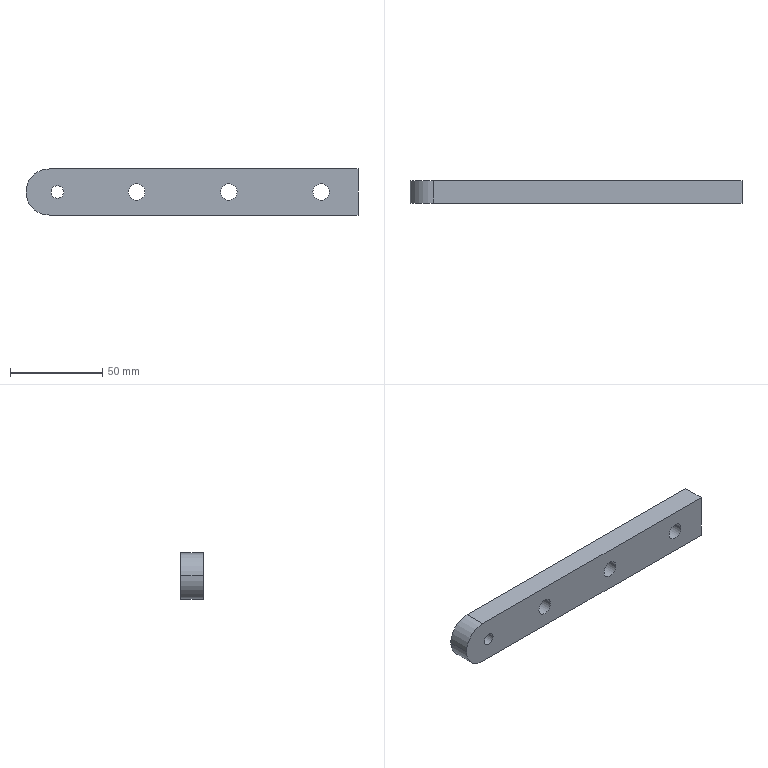Component | SolidWorks | CuttingDie-1_LocatingStrip-1 | 1 solid | 21 faces | box 180 x 12 x 25 mm | volume 49435 mm3 | cylinder 10 | cone 6 | plane 5 | commonest cylinder face diameters 9 x6 6.8 x2 25 x2
build123d program:
from build123d import *

# Parameters (mm, degrees)
SKETCH1_W                                         = 25
SKETCH1_H                                         = 12
BOSS_EXTRUDE1_DEPTH                               = 90
FILLET1_RADIUS                                    = 12.5
FILLET1_LENGTH                                    = 12
HOLE_SIZE_ACCORDING_TO_TYPE_1_OF_HEXA_D           = 9
HOLE_SIZE_ACCORDING_TO_TYPE_1_OF_HEXA_CSINK_D     = 17.6
HOLE_SIZE_ACCORDING_TO_TYPE_1_OF_HEXA_CSINK_ANGLE = 90
M8_TAPPED_HOLE1_D                                 = 6.8


with BuildPart() as part:
    # Sketch1 → Boss-Extrude1 (new, symmetric)
    with BuildSketch(Plane.XY):
        Rectangle(SKETCH1_W, SKETCH1_H)
    extrude(amount=BOSS_EXTRUDE1_DEPTH, both=True)

    # Fillet1: full round fillet: the end face becomes a half cylinder, R = half its width
    fillet1_face = Plane((0, 0, 90), x_dir=(0, 1, 0), z_dir=(0, 0, 1))  # on the end face: x along it, z out of the body
    fillet1_slab = fillet1_face.offset(-FILLET1_RADIUS / 2) * Box(FILLET1_LENGTH, 2 * FILLET1_RADIUS, FILLET1_RADIUS, mode=Mode.PRIVATE)  # the body's end, R deep
    fillet1_round = Plane((0, 0, 77.5), x_dir=(0, 0, 1), z_dir=(0, 1, 0)) * Cylinder(FILLET1_RADIUS, FILLET1_LENGTH, mode=Mode.PRIVATE)  # its axis R under the face
    add(fillet1_slab - fillet1_round, mode=Mode.SUBTRACT)

    # Hole Size _ according to_ Type 1 of Hexa (through all)
    with Locations(Plane(origin=(0, 6, 0), x_dir=(1, 0, 0), z_dir=(0, 1, 0))):
        with Locations((0, 70), (0, 20), (0, -30)):
            CounterSinkHole(HOLE_SIZE_ACCORDING_TO_TYPE_1_OF_HEXA_D / 2, HOLE_SIZE_ACCORDING_TO_TYPE_1_OF_HEXA_CSINK_D / 2, counter_sink_angle=HOLE_SIZE_ACCORDING_TO_TYPE_1_OF_HEXA_CSINK_ANGLE)

    # M8 Tapped Hole1 (through all)
    with Locations(Plane(origin=(0, 6, 0), x_dir=(1, 0, 0), z_dir=(0, 1, 0))):
        with Locations((0, -73)):
            Hole(M8_TAPPED_HOLE1_D / 2)


solid = part.part

# Placed as in the assembly
solid = solid.moved(Location((-441.772, -450.766, 1107), (0, -90, 0)))
STEP:
#1=COLOUR_RGB('',0.7922,0.8196,0.9333);
#2=FILL_AREA_STYLE_COLOUR('',#1);
#3=FILL_AREA_STYLE('',(#2));
#4=SURFACE_STYLE_FILL_AREA(#3);
#5=SURFACE_SIDE_STYLE('',(#4));
#6=SURFACE_STYLE_USAGE(.BOTH.,#5);
#7=PRESENTATION_STYLE_ASSIGNMENT((#6));
#8=CARTESIAN_POINT('',(-20.133,-17.983,43.583));
#9=VERTEX_POINT('',#8);
#10=CARTESIAN_POINT('',(-20.4,-17.983,43.583));
#11=VERTEX_POINT('',#10);
#12=CARTESIAN_POINT('',(-20.267,-17.983,43.583));
#13=DIRECTION('',(-0.,1.,0.));
#14=DIRECTION('',(-1.,0.,0.));
#15=AXIS2_PLACEMENT_3D('',#12,#13,#14);
#16=CIRCLE('',#15,0.1339);
#17=EDGE_CURVE('',#9,#11,#16,.T.);
#18=ORIENTED_EDGE('',*,*,#17,.F.);
#19=CARTESIAN_POINT('',(-20.133,-17.51,43.583));
#20=VERTEX_POINT('',#19);
#21=CARTESIAN_POINT('',(-20.133,-17.51,43.583));
#22=DIRECTION('',(-0.,1.,0.));
#23=VECTOR('',#22,39.37);
#24=LINE('',#21,#23);
#25=EDGE_CURVE('',#9,#20,#24,.T.);
#26=ORIENTED_EDGE('',*,*,#25,.T.);
#27=CARTESIAN_POINT('',(-20.4,-17.51,43.583));
#28=VERTEX_POINT('',#27);
#29=CARTESIAN_POINT('',(-20.267,-17.51,43.583));
#30=DIRECTION('',(-0.,1.,0.));
#31=DIRECTION('',(-1.,0.,0.));
#32=AXIS2_PLACEMENT_3D('',#29,#30,#31);
#33=CIRCLE('',#32,0.1339);
#34=EDGE_CURVE('',#20,#28,#33,.T.);
#35=ORIENTED_EDGE('',*,*,#34,.T.);
#36=CARTESIAN_POINT('',(-20.4,-17.51,43.583));
#37=DIRECTION('',(-0.,1.,0.));
#38=VECTOR('',#37,39.37);
#39=LINE('',#36,#38);
#40=EDGE_CURVE('',#11,#28,#39,.T.);
#41=ORIENTED_EDGE('',*,*,#40,.F.);
#42=EDGE_LOOP('',(#18,#26,#35,#41));
#43=FACE_OUTER_BOUND('',#42,.T.);
#44=CARTESIAN_POINT('',(-20.267,-17.51,43.583));
#45=DIRECTION('',(-0.,1.,0.));
#46=DIRECTION('',(-1.,0.,0.));
#47=AXIS2_PLACEMENT_3D('',#44,#45,#46);
#48=CYLINDRICAL_SURFACE('',#47,0.1339);
#49=ADVANCED_FACE('',(#43),#48,.F.);
#50=CARTESIAN_POINT('',(-14.46,-17.68,43.583));
#51=VERTEX_POINT('',#50);
#52=CARTESIAN_POINT('',(-14.814,-17.68,43.583));
#53=VERTEX_POINT('',#52);
#54=CARTESIAN_POINT('',(-14.637,-17.68,43.583));
#55=DIRECTION('',(-0.,1.,0.));
#56=DIRECTION('',(-1.,0.,0.));
#57=AXIS2_PLACEMENT_3D('',#54,#55,#56);
#58=CIRCLE('',#57,0.1772);
#59=EDGE_CURVE('',#51,#53,#58,.T.);
#60=ORIENTED_EDGE('',*,*,#59,.F.);
#61=CARTESIAN_POINT('',(-14.29,-17.51,43.583));
#62=VERTEX_POINT('',#61);
#63=CARTESIAN_POINT('',(-14.29,-17.51,43.583));
#64=DIRECTION('',(0.7071,0.7071,0.));
#65=VECTOR('',#64,39.37);
#66=LINE('',#63,#65);
#67=EDGE_CURVE('',#51,#62,#66,.T.);
#68=ORIENTED_EDGE('',*,*,#67,.T.);
#69=CARTESIAN_POINT('',(-14.983,-17.51,43.583));
#70=VERTEX_POINT('',#69);
#71=CARTESIAN_POINT('',(-14.637,-17.51,43.583));
#72=DIRECTION('',(-0.,1.,0.));
#73=DIRECTION('',(-1.,0.,0.));
#74=AXIS2_PLACEMENT_3D('',#71,#72,#73);
#75=CIRCLE('',#74,0.3465);
#76=EDGE_CURVE('',#62,#70,#75,.T.);
#77=ORIENTED_EDGE('',*,*,#76,.T.);
#78=CARTESIAN_POINT('',(-14.983,-17.51,43.583));
#79=DIRECTION('',(-0.7071,0.7071,-0.));
#80=VECTOR('',#79,39.37);
#81=LINE('',#78,#80);
#82=EDGE_CURVE('',#53,#70,#81,.T.);
#83=ORIENTED_EDGE('',*,*,#82,.F.);
#84=EDGE_LOOP('',(#60,#68,#77,#83));
#85=FACE_OUTER_BOUND('',#84,.T.);
#86=CARTESIAN_POINT('',(-14.637,-17.51,43.583));
#87=DIRECTION('',(-0.,1.,0.));
#88=DIRECTION('',(-1.,0.,0.));
#89=AXIS2_PLACEMENT_3D('',#86,#87,#88);
#90=CONICAL_SURFACE('',#89,0.3465,0.7854);
#91=ADVANCED_FACE('',(#85),#90,.F.);
#92=CARTESIAN_POINT('',(-14.46,-17.983,43.583));
#93=VERTEX_POINT('',#92);
#94=CARTESIAN_POINT('',(-14.814,-17.983,43.583));
#95=VERTEX_POINT('',#94);
#96=CARTESIAN_POINT('',(-14.637,-17.983,43.583));
#97=DIRECTION('',(-0.,1.,0.));
#98=DIRECTION('',(-1.,0.,0.));
#99=AXIS2_PLACEMENT_3D('',#96,#97,#98);
#100=CIRCLE('',#99,0.1772);
#101=EDGE_CURVE('',#93,#95,#100,.T.);
#102=ORIENTED_EDGE('',*,*,#101,.F.);
#103=CARTESIAN_POINT('',(-14.46,-17.51,43.583));
#104=DIRECTION('',(-0.,1.,0.));
#105=VECTOR('',#104,39.37);
#106=LINE('',#103,#105);
#107=EDGE_CURVE('',#93,#51,#106,.T.);
#108=ORIENTED_EDGE('',*,*,#107,.T.);
#109=ORIENTED_EDGE('',*,*,#59,.T.);
#110=CARTESIAN_POINT('',(-14.814,-17.51,43.583));
#111=DIRECTION('',(-0.,1.,0.));
#112=VECTOR('',#111,39.37);
#113=LINE('',#110,#112);
#114=EDGE_CURVE('',#95,#53,#113,.T.);
#115=ORIENTED_EDGE('',*,*,#114,.F.);
#116=EDGE_LOOP('',(#102,#108,#109,#115));
#117=FACE_OUTER_BOUND('',#116,.T.);
#118=CARTESIAN_POINT('',(-14.637,-17.51,43.583));
#119=DIRECTION('',(-0.,1.,0.));
#120=DIRECTION('',(-1.,0.,0.));
#121=AXIS2_PLACEMENT_3D('',#118,#119,#120);
#122=CYLINDRICAL_SURFACE('',#121,0.1772);
#123=ADVANCED_FACE('',(#117),#122,.F.);
#124=CARTESIAN_POINT('',(-16.428,-17.68,43.583));
#125=VERTEX_POINT('',#124);
#126=CARTESIAN_POINT('',(-16.782,-17.68,43.583));
#127=VERTEX_POINT('',#126);
#128=CARTESIAN_POINT('',(-16.605,-17.68,43.583));
#129=DIRECTION('',(-0.,1.,0.));
#130=DIRECTION('',(-1.,0.,0.));
#131=AXIS2_PLACEMENT_3D('',#128,#129,#130);
#132=CIRCLE('',#131,0.1772);
#133=EDGE_CURVE('',#125,#127,#132,.T.);
#134=ORIENTED_EDGE('',*,*,#133,.F.);
#135=CARTESIAN_POINT('',(-16.259,-17.51,43.583));
#136=VERTEX_POINT('',#135);
#137=CARTESIAN_POINT('',(-16.259,-17.51,43.583));
#138=DIRECTION('',(0.7071,0.7071,0.));
#139=VECTOR('',#138,39.37);
#140=LINE('',#137,#139);
#141=EDGE_CURVE('',#125,#136,#140,.T.);
#142=ORIENTED_EDGE('',*,*,#141,.T.);
#143=CARTESIAN_POINT('',(-16.952,-17.51,43.583));
#144=VERTEX_POINT('',#143);
#145=CARTESIAN_POINT('',(-16.605,-17.51,43.583));
#146=DIRECTION('',(-0.,1.,0.));
#147=DIRECTION('',(-1.,0.,0.));
#148=AXIS2_PLACEMENT_3D('',#145,#146,#147);
#149=CIRCLE('',#148,0.3465);
#150=EDGE_CURVE('',#136,#144,#149,.T.);
#151=ORIENTED_EDGE('',*,*,#150,.T.);
#152=CARTESIAN_POINT('',(-16.952,-17.51,43.583));
#153=DIRECTION('',(-0.7071,0.7071,-0.));
#154=VECTOR('',#153,39.37);
#155=LINE('',#152,#154);
#156=EDGE_CURVE('',#127,#144,#155,.T.);
#157=ORIENTED_EDGE('',*,*,#156,.F.);
#158=EDGE_LOOP('',(#134,#142,#151,#157));
#159=FACE_OUTER_BOUND('',#158,.T.);
#160=CARTESIAN_POINT('',(-16.605,-17.51,43.583));
#161=DIRECTION('',(-0.,1.,0.));
#162=DIRECTION('',(-1.,0.,0.));
#163=AXIS2_PLACEMENT_3D('',#160,#161,#162);
#164=CONICAL_SURFACE('',#163,0.3465,0.7854);
#165=ADVANCED_FACE('',(#159),#164,.F.);
#166=CARTESIAN_POINT('',(-16.428,-17.983,43.583));
#167=VERTEX_POINT('',#166);
#168=CARTESIAN_POINT('',(-16.782,-17.983,43.583));
#169=VERTEX_POINT('',#168);
#170=CARTESIAN_POINT('',(-16.605,-17.983,43.583));
#171=DIRECTION('',(-0.,1.,0.));
#172=DIRECTION('',(-1.,0.,0.));
#173=AXIS2_PLACEMENT_3D('',#170,#171,#172);
#174=CIRCLE('',#173,0.1772);
#175=EDGE_CURVE('',#167,#169,#174,.T.);
#176=ORIENTED_EDGE('',*,*,#175,.F.);
#177=CARTESIAN_POINT('',(-16.428,-17.51,43.583));
#178=DIRECTION('',(-0.,1.,0.));
#179=VECTOR('',#178,39.37);
#180=LINE('',#177,#179);
#181=EDGE_CURVE('',#167,#125,#180,.T.);
#182=ORIENTED_EDGE('',*,*,#181,.T.);
#183=ORIENTED_EDGE('',*,*,#133,.T.);
#184=CARTESIAN_POINT('',(-16.782,-17.51,43.583));
#185=DIRECTION('',(-0.,1.,0.));
#186=VECTOR('',#185,39.37);
#187=LINE('',#184,#186);
#188=EDGE_CURVE('',#169,#127,#187,.T.);
#189=ORIENTED_EDGE('',*,*,#188,.F.);
#190=EDGE_LOOP('',(#176,#182,#183,#189));
#191=FACE_OUTER_BOUND('',#190,.T.);
#192=CARTESIAN_POINT('',(-16.605,-17.51,43.583));
#193=DIRECTION('',(-0.,1.,0.));
#194=DIRECTION('',(-1.,0.,0.));
#195=AXIS2_PLACEMENT_3D('',#192,#193,#194);
#196=CYLINDRICAL_SURFACE('',#195,0.1772);
#197=ADVANCED_FACE('',(#191),#196,.F.);
#198=CARTESIAN_POINT('',(-18.397,-17.68,43.583));
#199=VERTEX_POINT('',#198);
#200=CARTESIAN_POINT('',(-18.751,-17.68,43.583));
#201=VERTEX_POINT('',#200);
#202=CARTESIAN_POINT('',(-18.574,-17.68,43.583));
#203=DIRECTION('',(-0.,1.,0.));
#204=DIRECTION('',(-1.,0.,0.));
#205=AXIS2_PLACEMENT_3D('',#202,#203,#204);
#206=CIRCLE('',#205,0.1772);
#207=EDGE_CURVE('',#199,#201,#206,.T.);
#208=ORIENTED_EDGE('',*,*,#207,.F.);
#209=CARTESIAN_POINT('',(-18.227,-17.51,43.583));
#210=VERTEX_POINT('',#209);
#211=CARTESIAN_POINT('',(-18.227,-17.51,43.583));
#212=DIRECTION('',(0.7071,0.7071,0.));
#213=VECTOR('',#212,39.37);
#214=LINE('',#211,#213);
#215=EDGE_CURVE('',#199,#210,#214,.T.);
#216=ORIENTED_EDGE('',*,*,#215,.T.);
#217=CARTESIAN_POINT('',(-18.92,-17.51,43.583));
#218=VERTEX_POINT('',#217);
#219=CARTESIAN_POINT('',(-18.574,-17.51,43.583));
#220=DIRECTION('',(-0.,1.,0.));
#221=DIRECTION('',(-1.,0.,0.));
#222=AXIS2_PLACEMENT_3D('',#219,#220,#221);
#223=CIRCLE('',#222,0.3465);
#224=EDGE_CURVE('',#210,#218,#223,.T.);
#225=ORIENTED_EDGE('',*,*,#224,.T.);
#226=CARTESIAN_POINT('',(-18.92,-17.51,43.583));
#227=DIRECTION('',(-0.7071,0.7071,-0.));
#228=VECTOR('',#227,39.37);
#229=LINE('',#226,#228);
#230=EDGE_CURVE('',#201,#218,#229,.T.);
#231=ORIENTED_EDGE('',*,*,#230,.F.);
#232=EDGE_LOOP('',(#208,#216,#225,#231));
#233=FACE_OUTER_BOUND('',#232,.T.);
#234=CARTESIAN_POINT('',(-18.574,-17.51,43.583));
#235=DIRECTION('',(-0.,1.,0.));
#236=DIRECTION('',(-1.,0.,0.));
#237=AXIS2_PLACEMENT_3D('',#234,#235,#236);
#238=CONICAL_SURFACE('',#237,0.3465,0.7854);
#239=ADVANCED_FACE('',(#233),#238,.F.);
#240=CARTESIAN_POINT('',(-18.397,-17.983,43.583));
#241=VERTEX_POINT('',#240);
#242=CARTESIAN_POINT('',(-18.751,-17.983,43.583));
#243=VERTEX_POINT('',#242);
#244=CARTESIAN_POINT('',(-18.574,-17.983,43.583));
#245=DIRECTION('',(-0.,1.,0.));
#246=DIRECTION('',(-1.,0.,0.));
#247=AXIS2_PLACEMENT_3D('',#244,#245,#246);
#248=CIRCLE('',#247,0.1772);
#249=EDGE_CURVE('',#241,#243,#248,.T.);
#250=ORIENTED_EDGE('',*,*,#249,.F.);
#251=CARTESIAN_POINT('',(-18.397,-17.51,43.583));
#252=DIRECTION('',(-0.,1.,0.));
#253=VECTOR('',#252,39.37);
#254=LINE('',#251,#253);
#255=EDGE_CURVE('',#241,#199,#254,.T.);
#256=ORIENTED_EDGE('',*,*,#255,.T.);
#257=ORIENTED_EDGE('',*,*,#207,.T.);
#258=CARTESIAN_POINT('',(-18.751,-17.51,43.583));
#259=DIRECTION('',(-0.,1.,0.));
#260=VECTOR('',#259,39.37);
#261=LINE('',#258,#260);
#262=EDGE_CURVE('',#243,#201,#261,.T.);
#263=ORIENTED_EDGE('',*,*,#262,.F.);
#264=EDGE_LOOP('',(#250,#256,#257,#263));
#265=FACE_OUTER_BOUND('',#264,.T.);
#266=CARTESIAN_POINT('',(-18.574,-17.51,43.583));
#267=DIRECTION('',(-0.,1.,0.));
#268=DIRECTION('',(-1.,0.,0.));
#269=AXIS2_PLACEMENT_3D('',#266,#267,#268);
#270=CYLINDRICAL_SURFACE('',#269,0.1772);
#271=ADVANCED_FACE('',(#265),#270,.F.);
#272=CARTESIAN_POINT('',(-20.936,-17.983,43.583));
#273=VERTEX_POINT('',#272);
#274=CARTESIAN_POINT('',(-20.444,-17.983,43.091));
#275=VERTEX_POINT('',#274);
#276=CARTESIAN_POINT('',(-20.444,-17.983,43.583));
#277=DIRECTION('',(0.,-1.,0.));
#278=DIRECTION('',(0.,0.,-1.));
#279=AXIS2_PLACEMENT_3D('',#276,#277,#278);
#280=CIRCLE('',#279,0.4921);
#281=EDGE_CURVE('',#273,#275,#280,.T.);
#282=ORIENTED_EDGE('',*,*,#281,.F.);
#283=CARTESIAN_POINT('',(-20.936,-17.51,43.583));
#284=VERTEX_POINT('',#283);
#285=CARTESIAN_POINT('',(-20.936,-17.51,43.583));
#286=DIRECTION('',(-0.,1.,0.));
#287=VECTOR('',#286,39.37);
#288=LINE('',#285,#287);
#289=EDGE_CURVE('',#273,#284,#288,.T.);
#290=ORIENTED_EDGE('',*,*,#289,.T.);
#291=CARTESIAN_POINT('',(-20.444,-17.51,43.091));
#292=VERTEX_POINT('',#291);
#293=CARTESIAN_POINT('',(-20.444,-17.51,43.583));
#294=DIRECTION('',(-0.,1.,0.));
#295=DIRECTION('',(1.,0.,0.));
#296=AXIS2_PLACEMENT_3D('',#293,#294,#295);
#297=CIRCLE('',#296,0.4921);
#298=EDGE_CURVE('',#292,#284,#297,.T.);
#299=ORIENTED_EDGE('',*,*,#298,.F.);
#300=CARTESIAN_POINT('',(-20.444,-17.51,43.091));
#301=DIRECTION('',(-0.,1.,0.));
#302=VECTOR('',#301,39.37);
#303=LINE('',#300,#302);
#304=EDGE_CURVE('',#275,#292,#303,.T.);
#305=ORIENTED_EDGE('',*,*,#304,.F.);
#306=EDGE_LOOP('',(#282,#290,#299,#305));
#307=FACE_OUTER_BOUND('',#306,.T.);
#308=CARTESIAN_POINT('',(-20.444,-17.51,43.583));
#309=DIRECTION('',(-0.,1.,0.));
#310=DIRECTION('',(-1.,0.,0.));
#311=AXIS2_PLACEMENT_3D('',#308,#309,#310);
#312=CYLINDRICAL_SURFACE('',#311,0.4921);
#313=ADVANCED_FACE('',(#307),#312,.T.);
#314=ORIENTED_EDGE('',*,*,#289,.F.);
#315=CARTESIAN_POINT('',(-20.444,-17.983,44.075));
#316=VERTEX_POINT('',#315);
#317=CARTESIAN_POINT('',(-20.444,-17.983,43.583));
#318=DIRECTION('',(0.,-1.,0.));
#319=DIRECTION('',(0.,0.,-1.));
#320=AXIS2_PLACEMENT_3D('',#317,#318,#319);
#321=CIRCLE('',#320,0.4921);
#322=EDGE_CURVE('',#316,#273,#321,.T.);
#323=ORIENTED_EDGE('',*,*,#322,.F.);
#324=CARTESIAN_POINT('',(-20.444,-17.51,44.075));
#325=VERTEX_POINT('',#324);
#326=CARTESIAN_POINT('',(-20.444,-17.51,44.075));
#327=DIRECTION('',(0.,-1.,-0.));
#328=VECTOR('',#327,39.37);
#329=LINE('',#326,#328);
#330=EDGE_CURVE('',#325,#316,#329,.T.);
#331=ORIENTED_EDGE('',*,*,#330,.F.);
#332=CARTESIAN_POINT('',(-20.444,-17.51,43.583));
#333=DIRECTION('',(-0.,1.,0.));
#334=DIRECTION('',(1.,0.,0.));
#335=AXIS2_PLACEMENT_3D('',#332,#333,#334);
#336=CIRCLE('',#335,0.4921);
#337=EDGE_CURVE('',#284,#325,#336,.T.);
#338=ORIENTED_EDGE('',*,*,#337,.F.);
#339=EDGE_LOOP('',(#314,#323,#331,#338));
#340=FACE_OUTER_BOUND('',#339,.T.);
#341=CARTESIAN_POINT('',(-20.444,-17.51,43.583));
#342=DIRECTION('',(-0.,1.,0.));
#343=DIRECTION('',(-1.,0.,0.));
#344=AXIS2_PLACEMENT_3D('',#341,#342,#343);
#345=CYLINDRICAL_SURFACE('',#344,0.4921);
#346=ADVANCED_FACE('',(#340),#345,.T.);
#347=CARTESIAN_POINT('',(-13.849,-17.983,43.091));
#348=VERTEX_POINT('',#347);
#349=CARTESIAN_POINT('',(-20.936,-17.983,43.091));
#350=DIRECTION('',(1.,0.,0.));
#351=VECTOR('',#350,39.37);
#352=LINE('',#349,#351);
#353=EDGE_CURVE('',#275,#348,#352,.T.);
#354=ORIENTED_EDGE('',*,*,#353,.F.);
#355=ORIENTED_EDGE('',*,*,#304,.T.);
#356=CARTESIAN_POINT('',(-13.849,-17.51,43.091));
#357=VERTEX_POINT('',#356);
#358=CARTESIAN_POINT('',(-20.936,-17.51,43.091));
#359=DIRECTION('',(1.,0.,0.));
#360=VECTOR('',#359,39.37);
#361=LINE('',#358,#360);
#362=EDGE_CURVE('',#292,#357,#361,.T.);
#363=ORIENTED_EDGE('',*,*,#362,.T.);
#364=CARTESIAN_POINT('',(-13.849,-17.983,43.091));
#365=DIRECTION('',(0.,-1.,-0.));
#366=VECTOR('',#365,39.37);
#367=LINE('',#364,#366);
#368=EDGE_CURVE('',#357,#348,#367,.T.);
#369=ORIENTED_EDGE('',*,*,#368,.T.);
#370=EDGE_LOOP('',(#354,#355,#363,#369));
#371=FACE_OUTER_BOUND('',#370,.T.);
#372=CARTESIAN_POINT('',(-20.936,-17.983,43.091));
#373=DIRECTION('',(-0.,-0.,1.));
#374=DIRECTION('',(1.,0.,0.));
#375=AXIS2_PLACEMENT_3D('',#372,#373,#374);
#376=PLANE('',#375);
#377=ADVANCED_FACE('',(#371),#376,.F.);
#378=CARTESIAN_POINT('',(-20.267,-17.983,43.583));
#379=DIRECTION('',(-0.,1.,0.));
#380=DIRECTION('',(-1.,0.,0.));
#381=AXIS2_PLACEMENT_3D('',#378,#379,#380);
#382=CIRCLE('',#381,0.1339);
#383=EDGE_CURVE('',#11,#9,#382,.T.);
#384=ORIENTED_EDGE('',*,*,#383,.T.);
#385=ORIENTED_EDGE('',*,*,#17,.T.);
#386=EDGE_LOOP('',(#384,#385));
#387=FACE_BOUND('',#386,.T.);
#388=CARTESIAN_POINT('',(-14.637,-17.983,43.583));
#389=DIRECTION('',(-0.,1.,0.));
#390=DIRECTION('',(-1.,0.,0.));
#391=AXIS2_PLACEMENT_3D('',#388,#389,#390);
#392=CIRCLE('',#391,0.1772);
#393=EDGE_CURVE('',#95,#93,#392,.T.);
#394=ORIENTED_EDGE('',*,*,#393,.T.);
#395=ORIENTED_EDGE('',*,*,#101,.T.);
#396=EDGE_LOOP('',(#394,#395));
#397=FACE_BOUND('',#396,.T.);
#398=CARTESIAN_POINT('',(-16.605,-17.983,43.583));
#399=DIRECTION('',(-0.,1.,0.));
#400=DIRECTION('',(-1.,0.,0.));
#401=AXIS2_PLACEMENT_3D('',#398,#399,#400);
#402=CIRCLE('',#401,0.1772);
#403=EDGE_CURVE('',#169,#167,#402,.T.);
#404=ORIENTED_EDGE('',*,*,#403,.T.);
#405=ORIENTED_EDGE('',*,*,#175,.T.);
#406=EDGE_LOOP('',(#404,#405));
#407=FACE_BOUND('',#406,.T.);
#408=CARTESIAN_POINT('',(-18.574,-17.983,43.583));
#409=DIRECTION('',(-0.,1.,0.));
#410=DIRECTION('',(-1.,0.,0.));
#411=AXIS2_PLACEMENT_3D('',#408,#409,#410);
#412=CIRCLE('',#411,0.1772);
#413=EDGE_CURVE('',#243,#241,#412,.T.);
#414=ORIENTED_EDGE('',*,*,#413,.T.);
#415=ORIENTED_EDGE('',*,*,#249,.T.);
#416=EDGE_LOOP('',(#414,#415));
#417=FACE_BOUND('',#416,.T.);
#418=CARTESIAN_POINT('',(-13.849,-17.983,44.075));
#419=VERTEX_POINT('',#418);
#420=CARTESIAN_POINT('',(-20.936,-17.983,44.075));
#421=DIRECTION('',(1.,0.,0.));
#422=VECTOR('',#421,39.37);
#423=LINE('',#420,#422);
#424=EDGE_CURVE('',#316,#419,#423,.T.);
#425=ORIENTED_EDGE('',*,*,#424,.F.);
#426=ORIENTED_EDGE('',*,*,#322,.T.);
#427=ORIENTED_EDGE('',*,*,#281,.T.);
#428=ORIENTED_EDGE('',*,*,#353,.T.);
#429=CARTESIAN_POINT('',(-13.849,-17.983,44.075));
#430=DIRECTION('',(-0.,0.,1.));
#431=VECTOR('',#430,39.37);
#432=LINE('',#429,#431);
#433=EDGE_CURVE('',#348,#419,#432,.T.);
#434=ORIENTED_EDGE('',*,*,#433,.T.);
#435=EDGE_LOOP('',(#425,#426,#427,#428,#434));
#436=FACE_OUTER_BOUND('',#435,.T.);
#437=CARTESIAN_POINT('',(-20.936,-17.983,44.075));
#438=DIRECTION('',(-0.,1.,-0.));
#439=DIRECTION('',(0.,-0.,-1.));
#440=AXIS2_PLACEMENT_3D('',#437,#438,#439);
#441=PLANE('',#440);
#442=ADVANCED_FACE('',(#387,#397,#407,#417,#436),#441,.F.);
#443=CARTESIAN_POINT('',(-13.849,-17.51,44.075));
#444=VERTEX_POINT('',#443);
#445=CARTESIAN_POINT('',(-20.936,-17.51,44.075));
#446=DIRECTION('',(1.,0.,0.));
#447=VECTOR('',#446,39.37);
#448=LINE('',#445,#447);
#449=EDGE_CURVE('',#325,#444,#448,.T.);
#450=ORIENTED_EDGE('',*,*,#449,.F.);
#451=ORIENTED_EDGE('',*,*,#330,.T.);
#452=ORIENTED_EDGE('',*,*,#424,.T.);
#453=CARTESIAN_POINT('',(-13.849,-17.983,44.075));
#454=DIRECTION('',(-0.,1.,0.));
#455=VECTOR('',#454,39.37);
#456=LINE('',#453,#455);
#457=EDGE_CURVE('',#419,#444,#456,.T.);
#458=ORIENTED_EDGE('',*,*,#457,.T.);
#459=EDGE_LOOP('',(#450,#451,#452,#458));
#460=FACE_OUTER_BOUND('',#459,.T.);
#461=CARTESIAN_POINT('',(-20.936,-17.983,44.075));
#462=DIRECTION('',(0.,0.,-1.));
#463=DIRECTION('',(-1.,-0.,-0.));
#464=AXIS2_PLACEMENT_3D('',#461,#462,#463);
#465=PLANE('',#464);
#466=ADVANCED_FACE('',(#460),#465,.F.);
#467=CARTESIAN_POINT('',(-20.267,-17.51,43.583));
#468=DIRECTION('',(-0.,1.,0.));
#469=DIRECTION('',(-1.,0.,0.));
#470=AXIS2_PLACEMENT_3D('',#467,#468,#469);
#471=CIRCLE('',#470,0.1339);
#472=EDGE_CURVE('',#28,#20,#471,.T.);
#473=ORIENTED_EDGE('',*,*,#472,.F.);
#474=ORIENTED_EDGE('',*,*,#34,.F.);
#475=EDGE_LOOP('',(#473,#474));
#476=FACE_BOUND('',#475,.T.);
#477=CARTESIAN_POINT('',(-14.637,-17.51,43.583));
#478=DIRECTION('',(-0.,1.,0.));
#479=DIRECTION('',(-1.,0.,0.));
#480=AXIS2_PLACEMENT_3D('',#477,#478,#479);
#481=CIRCLE('',#480,0.3465);
#482=EDGE_CURVE('',#70,#62,#481,.T.);
#483=ORIENTED_EDGE('',*,*,#482,.F.);
#484=ORIENTED_EDGE('',*,*,#76,.F.);
#485=EDGE_LOOP('',(#483,#484));
#486=FACE_BOUND('',#485,.T.);
#487=CARTESIAN_POINT('',(-16.605,-17.51,43.583));
#488=DIRECTION('',(-0.,1.,0.));
#489=DIRECTION('',(-1.,0.,0.));
#490=AXIS2_PLACEMENT_3D('',#487,#488,#489);
#491=CIRCLE('',#490,0.3465);
#492=EDGE_CURVE('',#144,#136,#491,.T.);
#493=ORIENTED_EDGE('',*,*,#492,.F.);
#494=ORIENTED_EDGE('',*,*,#150,.F.);
#495=EDGE_LOOP('',(#493,#494));
#496=FACE_BOUND('',#495,.T.);
#497=CARTESIAN_POINT('',(-18.574,-17.51,43.583));
#498=DIRECTION('',(-0.,1.,0.));
#499=DIRECTION('',(-1.,0.,0.));
#500=AXIS2_PLACEMENT_3D('',#497,#498,#499);
#501=CIRCLE('',#500,0.3465);
#502=EDGE_CURVE('',#218,#210,#501,.T.);
#503=ORIENTED_EDGE('',*,*,#502,.F.);
#504=ORIENTED_EDGE('',*,*,#224,.F.);
#505=EDGE_LOOP('',(#503,#504));
#506=FACE_BOUND('',#505,.T.);
#507=ORIENTED_EDGE('',*,*,#362,.F.);
#508=ORIENTED_EDGE('',*,*,#298,.T.);
#509=ORIENTED_EDGE('',*,*,#337,.T.);
#510=ORIENTED_EDGE('',*,*,#449,.T.);
#511=CARTESIAN_POINT('',(-13.849,-17.51,44.075));
#512=DIRECTION('',(0.,0.,-1.));
#513=VECTOR('',#512,39.37);
#514=LINE('',#511,#513);
#515=EDGE_CURVE('',#444,#357,#514,.T.);
#516=ORIENTED_EDGE('',*,*,#515,.T.);
#517=EDGE_LOOP('',(#507,#508,#509,#510,#516));
#518=FACE_OUTER_BOUND('',#517,.T.);
#519=CARTESIAN_POINT('',(-20.936,-17.51,44.075));
#520=DIRECTION('',(0.,-1.,-0.));
#521=DIRECTION('',(1.,0.,0.));
#522=AXIS2_PLACEMENT_3D('',#519,#520,#521);
#523=PLANE('',#522);
#524=ADVANCED_FACE('',(#476,#486,#496,#506,#518),#523,.F.);
#525=ORIENTED_EDGE('',*,*,#368,.F.);
#526=ORIENTED_EDGE('',*,*,#515,.F.);
#527=ORIENTED_EDGE('',*,*,#457,.F.);
#528=ORIENTED_EDGE('',*,*,#433,.F.);
#529=EDGE_LOOP('',(#525,#526,#527,#528));
#530=FACE_OUTER_BOUND('',#529,.T.);
#531=CARTESIAN_POINT('',(-13.849,-17.747,43.583));
#532=DIRECTION('',(-1.,-0.,-0.));
#533=DIRECTION('',(-0.,-0.,1.));
#534=AXIS2_PLACEMENT_3D('',#531,#532,#533);
#535=PLANE('',#534);
#536=ADVANCED_FACE('',(#530),#535,.F.);
#537=ORIENTED_EDGE('',*,*,#255,.F.);
#538=ORIENTED_EDGE('',*,*,#413,.F.);
#539=ORIENTED_EDGE('',*,*,#262,.T.);
#540=CARTESIAN_POINT('',(-18.574,-17.68,43.583));
#541=DIRECTION('',(-0.,1.,0.));
#542=DIRECTION('',(-1.,0.,0.));
#543=AXIS2_PLACEMENT_3D('',#540,#541,#542);
#544=CIRCLE('',#543,0.1772);
#545=EDGE_CURVE('',#201,#199,#544,.T.);
#546=ORIENTED_EDGE('',*,*,#545,.T.);
#547=EDGE_LOOP('',(#537,#538,#539,#546));
#548=FACE_OUTER_BOUND('',#547,.T.);
#549=CARTESIAN_POINT('',(-18.574,-17.51,43.583));
#550=DIRECTION('',(-0.,1.,0.));
#551=DIRECTION('',(-1.,0.,0.));
#552=AXIS2_PLACEMENT_3D('',#549,#550,#551);
#553=CYLINDRICAL_SURFACE('',#552,0.1772);
#554=ADVANCED_FACE('',(#548),#553,.F.);
#555=ORIENTED_EDGE('',*,*,#215,.F.);
#556=ORIENTED_EDGE('',*,*,#545,.F.);
#557=ORIENTED_EDGE('',*,*,#230,.T.);
#558=ORIENTED_EDGE('',*,*,#502,.T.);
#559=EDGE_LOOP('',(#555,#556,#557,#558));
#560=FACE_OUTER_BOUND('',#559,.T.);
#561=CARTESIAN_POINT('',(-18.574,-17.51,43.583));
#562=DIRECTION('',(-0.,1.,0.));
#563=DIRECTION('',(-1.,0.,0.));
#564=AXIS2_PLACEMENT_3D('',#561,#562,#563);
#565=CONICAL_SURFACE('',#564,0.3465,0.7854);
#566=ADVANCED_FACE('',(#560),#565,.F.);
#567=ORIENTED_EDGE('',*,*,#181,.F.);
#568=ORIENTED_EDGE('',*,*,#403,.F.);
#569=ORIENTED_EDGE('',*,*,#188,.T.);
#570=CARTESIAN_POINT('',(-16.605,-17.68,43.583));
#571=DIRECTION('',(-0.,1.,0.));
#572=DIRECTION('',(-1.,0.,0.));
#573=AXIS2_PLACEMENT_3D('',#570,#571,#572);
#574=CIRCLE('',#573,0.1772);
#575=EDGE_CURVE('',#127,#125,#574,.T.);
#576=ORIENTED_EDGE('',*,*,#575,.T.);
#577=EDGE_LOOP('',(#567,#568,#569,#576));
#578=FACE_OUTER_BOUND('',#577,.T.);
#579=CARTESIAN_POINT('',(-16.605,-17.51,43.583));
#580=DIRECTION('',(-0.,1.,0.));
#581=DIRECTION('',(-1.,0.,0.));
#582=AXIS2_PLACEMENT_3D('',#579,#580,#581);
#583=CYLINDRICAL_SURFACE('',#582,0.1772);
#584=ADVANCED_FACE('',(#578),#583,.F.);
#585=ORIENTED_EDGE('',*,*,#141,.F.);
#586=ORIENTED_EDGE('',*,*,#575,.F.);
#587=ORIENTED_EDGE('',*,*,#156,.T.);
#588=ORIENTED_EDGE('',*,*,#492,.T.);
#589=EDGE_LOOP('',(#585,#586,#587,#588));
#590=FACE_OUTER_BOUND('',#589,.T.);
#591=CARTESIAN_POINT('',(-16.605,-17.51,43.583));
#592=DIRECTION('',(-0.,1.,0.));
#593=DIRECTION('',(-1.,0.,0.));
#594=AXIS2_PLACEMENT_3D('',#591,#592,#593);
#595=CONICAL_SURFACE('',#594,0.3465,0.7854);
#596=ADVANCED_FACE('',(#590),#595,.F.);
#597=ORIENTED_EDGE('',*,*,#107,.F.);
#598=ORIENTED_EDGE('',*,*,#393,.F.);
#599=ORIENTED_EDGE('',*,*,#114,.T.);
#600=CARTESIAN_POINT('',(-14.637,-17.68,43.583));
#601=DIRECTION('',(-0.,1.,0.));
#602=DIRECTION('',(-1.,0.,0.));
#603=AXIS2_PLACEMENT_3D('',#600,#601,#602);
#604=CIRCLE('',#603,0.1772);
#605=EDGE_CURVE('',#53,#51,#604,.T.);
#606=ORIENTED_EDGE('',*,*,#605,.T.);
#607=EDGE_LOOP('',(#597,#598,#599,#606));
#608=FACE_OUTER_BOUND('',#607,.T.);
#609=CARTESIAN_POINT('',(-14.637,-17.51,43.583));
#610=DIRECTION('',(-0.,1.,0.));
#611=DIRECTION('',(-1.,0.,0.));
#612=AXIS2_PLACEMENT_3D('',#609,#610,#611);
#613=CYLINDRICAL_SURFACE('',#612,0.1772);
#614=ADVANCED_FACE('',(#608),#613,.F.);
#615=ORIENTED_EDGE('',*,*,#67,.F.);
#616=ORIENTED_EDGE('',*,*,#605,.F.);
#617=ORIENTED_EDGE('',*,*,#82,.T.);
#618=ORIENTED_EDGE('',*,*,#482,.T.);
#619=EDGE_LOOP('',(#615,#616,#617,#618));
#620=FACE_OUTER_BOUND('',#619,.T.);
#621=CARTESIAN_POINT('',(-14.637,-17.51,43.583));
#622=DIRECTION('',(-0.,1.,0.));
#623=DIRECTION('',(-1.,0.,0.));
#624=AXIS2_PLACEMENT_3D('',#621,#622,#623);
#625=CONICAL_SURFACE('',#624,0.3465,0.7854);
#626=ADVANCED_FACE('',(#620),#625,.F.);
#627=ORIENTED_EDGE('',*,*,#25,.F.);
#628=ORIENTED_EDGE('',*,*,#383,.F.);
#629=ORIENTED_EDGE('',*,*,#40,.T.);
#630=ORIENTED_EDGE('',*,*,#472,.T.);
#631=EDGE_LOOP('',(#627,#628,#629,#630));
#632=FACE_OUTER_BOUND('',#631,.T.);
#633=CARTESIAN_POINT('',(-20.267,-17.51,43.583));
#634=DIRECTION('',(-0.,1.,0.));
#635=DIRECTION('',(-1.,0.,0.));
#636=AXIS2_PLACEMENT_3D('',#633,#634,#635);
#637=CYLINDRICAL_SURFACE('',#636,0.1339);
#638=ADVANCED_FACE('',(#632),#637,.F.);
#639=CLOSED_SHELL('',(#49,#91,#123,#165,#197,#239,#271,#313,#346,#377,#442,#466,#524,#536,#554,#566,#584,#596,#614,#626,#638));
#640=MANIFOLD_SOLID_BREP('',#639);
#641=STYLED_ITEM('',(#7),#640);
#642=(LENGTH_UNIT()NAMED_UNIT(*)SI_UNIT($,.METRE.));
#643=LENGTH_MEASURE_WITH_UNIT(LENGTH_MEASURE(0.0254),#642);
#644=DIMENSIONAL_EXPONENTS(1.,0.,0.,0.,0.,0.,0.);
#645=(CONVERSION_BASED_UNIT('',#643)LENGTH_UNIT()NAMED_UNIT(#644));
#646=UNCERTAINTY_MEASURE_WITH_UNIT(LENGTH_MEASURE(0.00001),#645,'','');
#647=(NAMED_UNIT(*)PLANE_ANGLE_UNIT()SI_UNIT($,.RADIAN.));
#648=(NAMED_UNIT(*)SI_UNIT($,.STERADIAN.)SOLID_ANGLE_UNIT());
#649=(GEOMETRIC_REPRESENTATION_CONTEXT(3)GLOBAL_UNCERTAINTY_ASSIGNED_CONTEXT((#646))GLOBAL_UNIT_ASSIGNED_CONTEXT((#645,#647,#648))REPRESENTATION_CONTEXT('',''));
#650=MECHANICAL_DESIGN_GEOMETRIC_PRESENTATION_REPRESENTATION('',(#641),#649);
#651=PRESENTATION_LAYER_ASSIGNMENT('','',(#641));
#652=CARTESIAN_POINT('',(0.,0.,0.));
#653=DIRECTION('',(0.,0.,1.));
#654=DIRECTION('',(1.,0.,0.));
#655=AXIS2_PLACEMENT_3D('',#652,#653,#654);
#656=(LENGTH_UNIT()NAMED_UNIT(*)SI_UNIT($,.METRE.));
#657=LENGTH_MEASURE_WITH_UNIT(LENGTH_MEASURE(0.0254),#656);
#658=DIMENSIONAL_EXPONENTS(1.,0.,0.,0.,0.,0.,0.);
#659=(CONVERSION_BASED_UNIT('',#657)LENGTH_UNIT()NAMED_UNIT(#658));
#660=UNCERTAINTY_MEASURE_WITH_UNIT(LENGTH_MEASURE(0.00001),#659,'','');
#661=(NAMED_UNIT(*)PLANE_ANGLE_UNIT()SI_UNIT($,.RADIAN.));
#662=(NAMED_UNIT(*)SI_UNIT($,.STERADIAN.)SOLID_ANGLE_UNIT());
#663=(GEOMETRIC_REPRESENTATION_CONTEXT(3)GLOBAL_UNCERTAINTY_ASSIGNED_CONTEXT((#660))GLOBAL_UNIT_ASSIGNED_CONTEXT((#659,#661,#662))REPRESENTATION_CONTEXT('',''));
#664=ADVANCED_BREP_SHAPE_REPRESENTATION('',(#640,#655),#663);